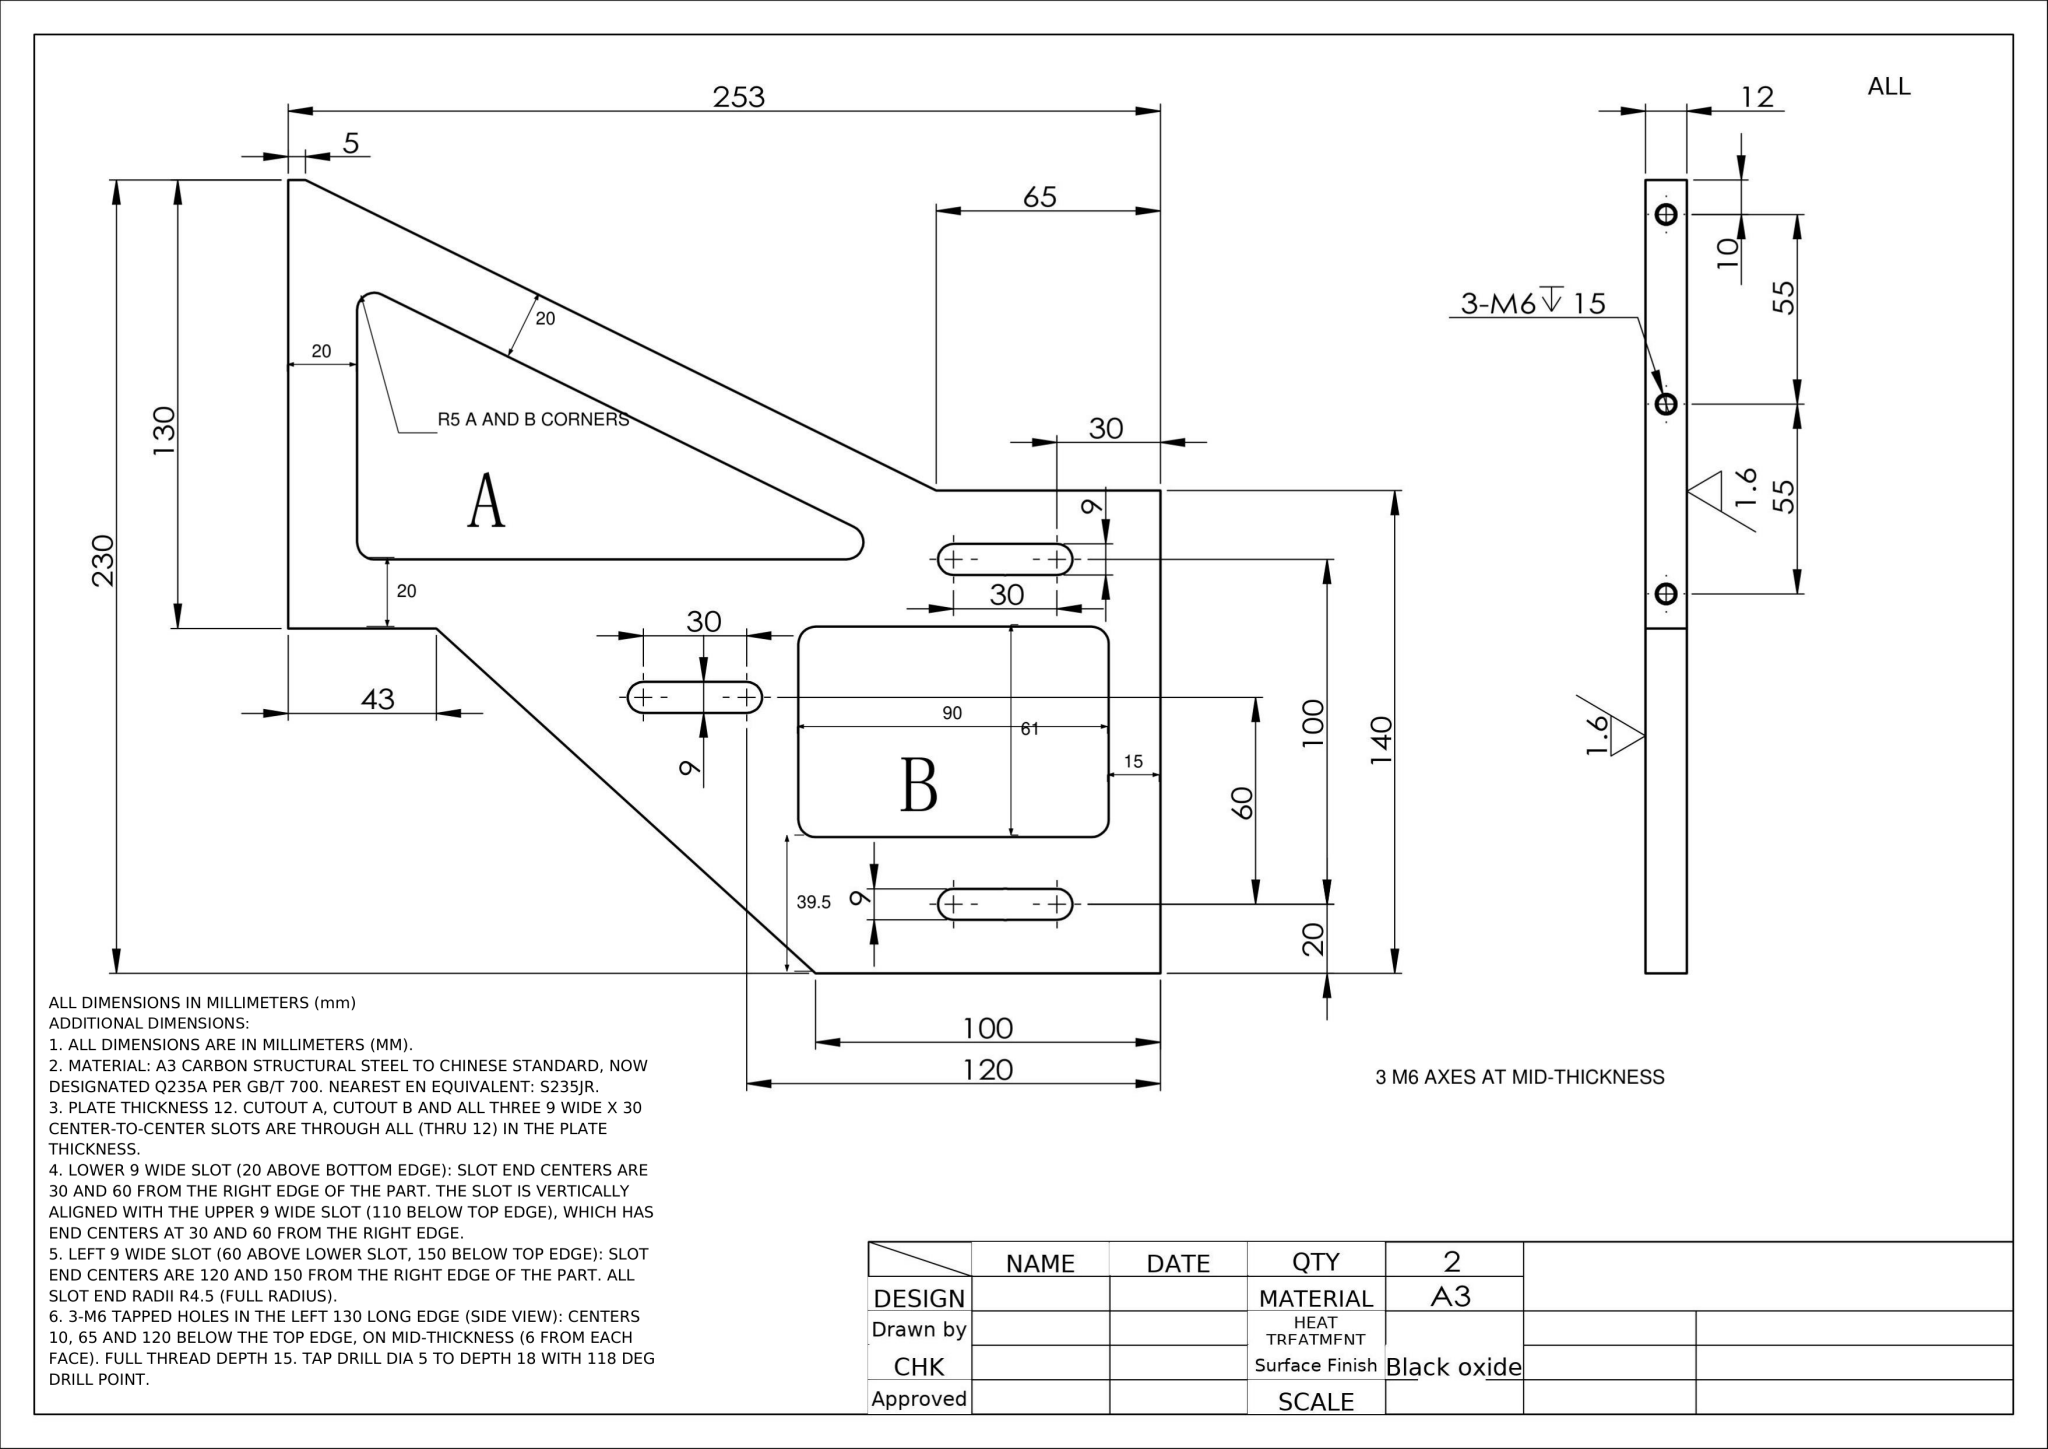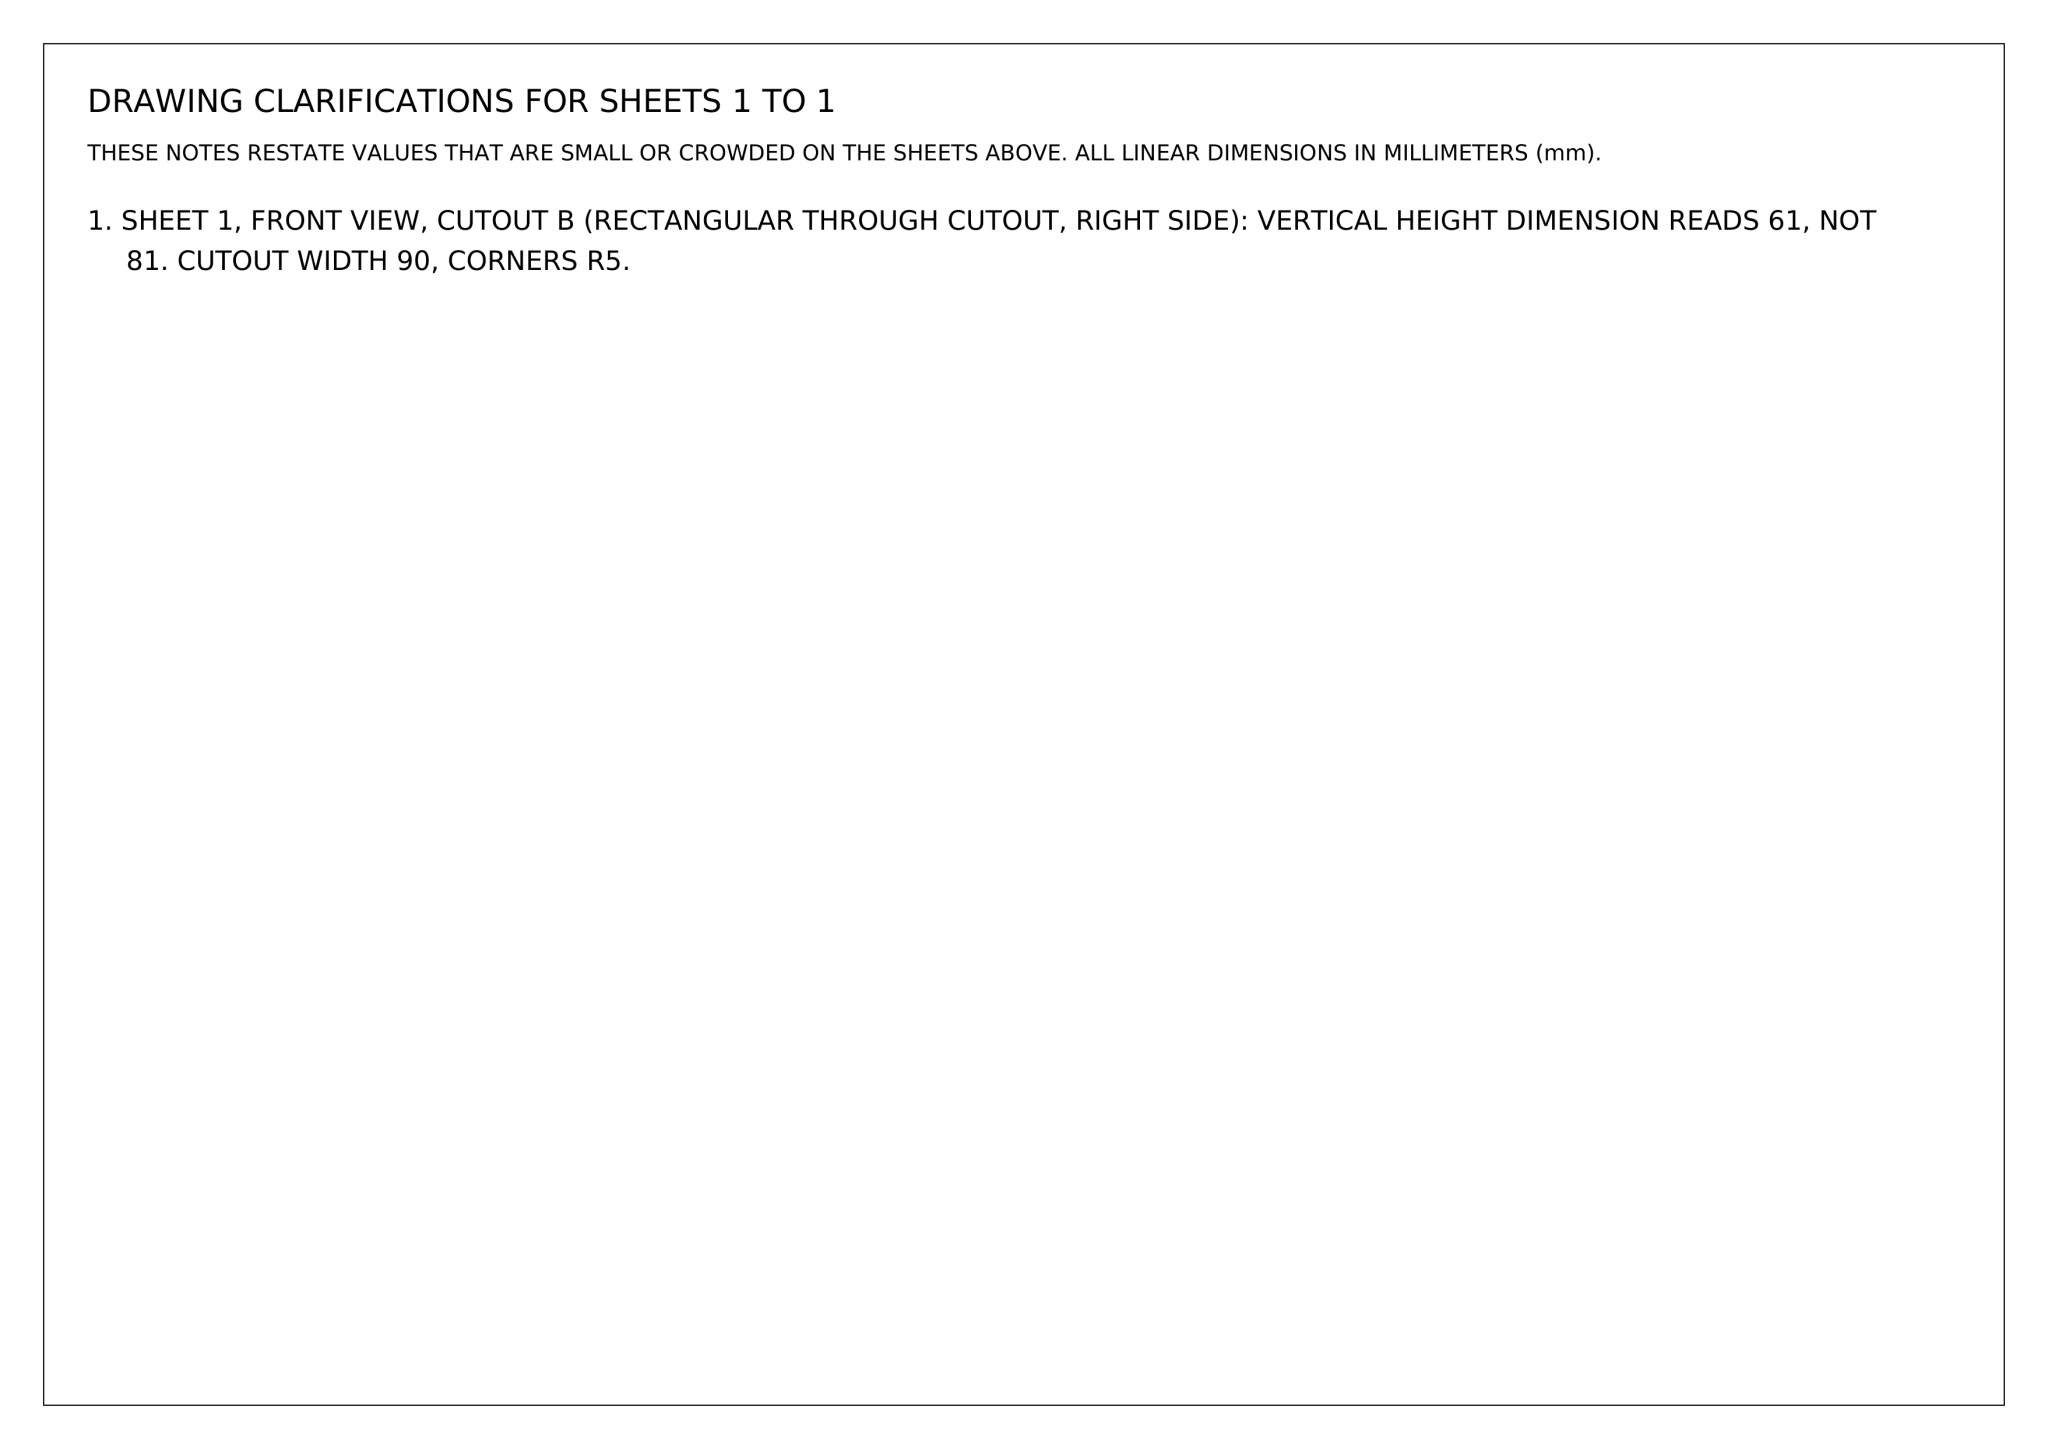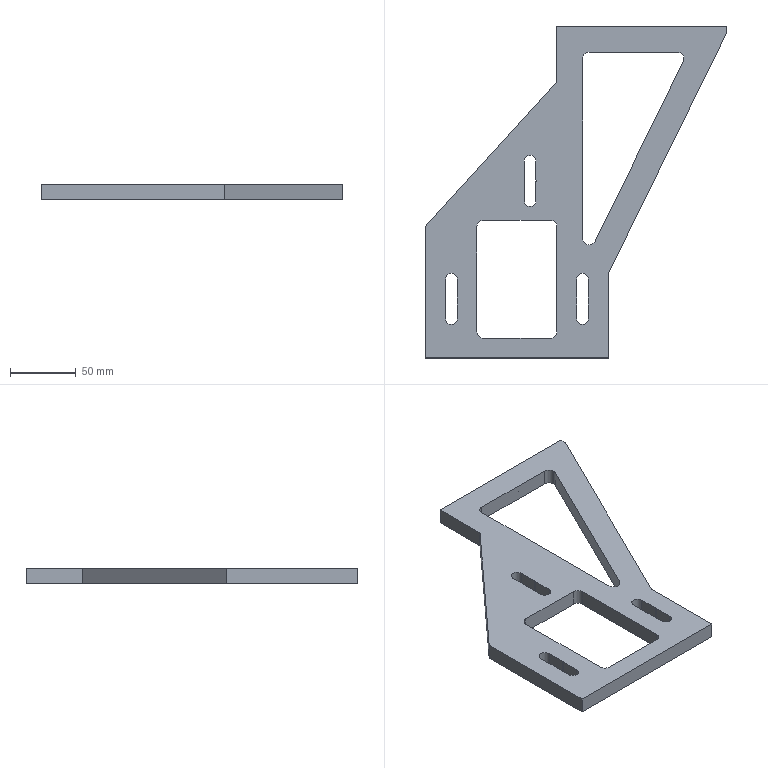Part | NX | mm | Triangular Perforated Mounting Plate | 1 solid | 73 faces | box 230 x 253 x 12 mm | volume 254939 mm3 | cylinder 35 | plane 32 | cone 6 | commonest cylinder face diameters 9.1 x9 10 x8 5 x6 6 x6 9 x6